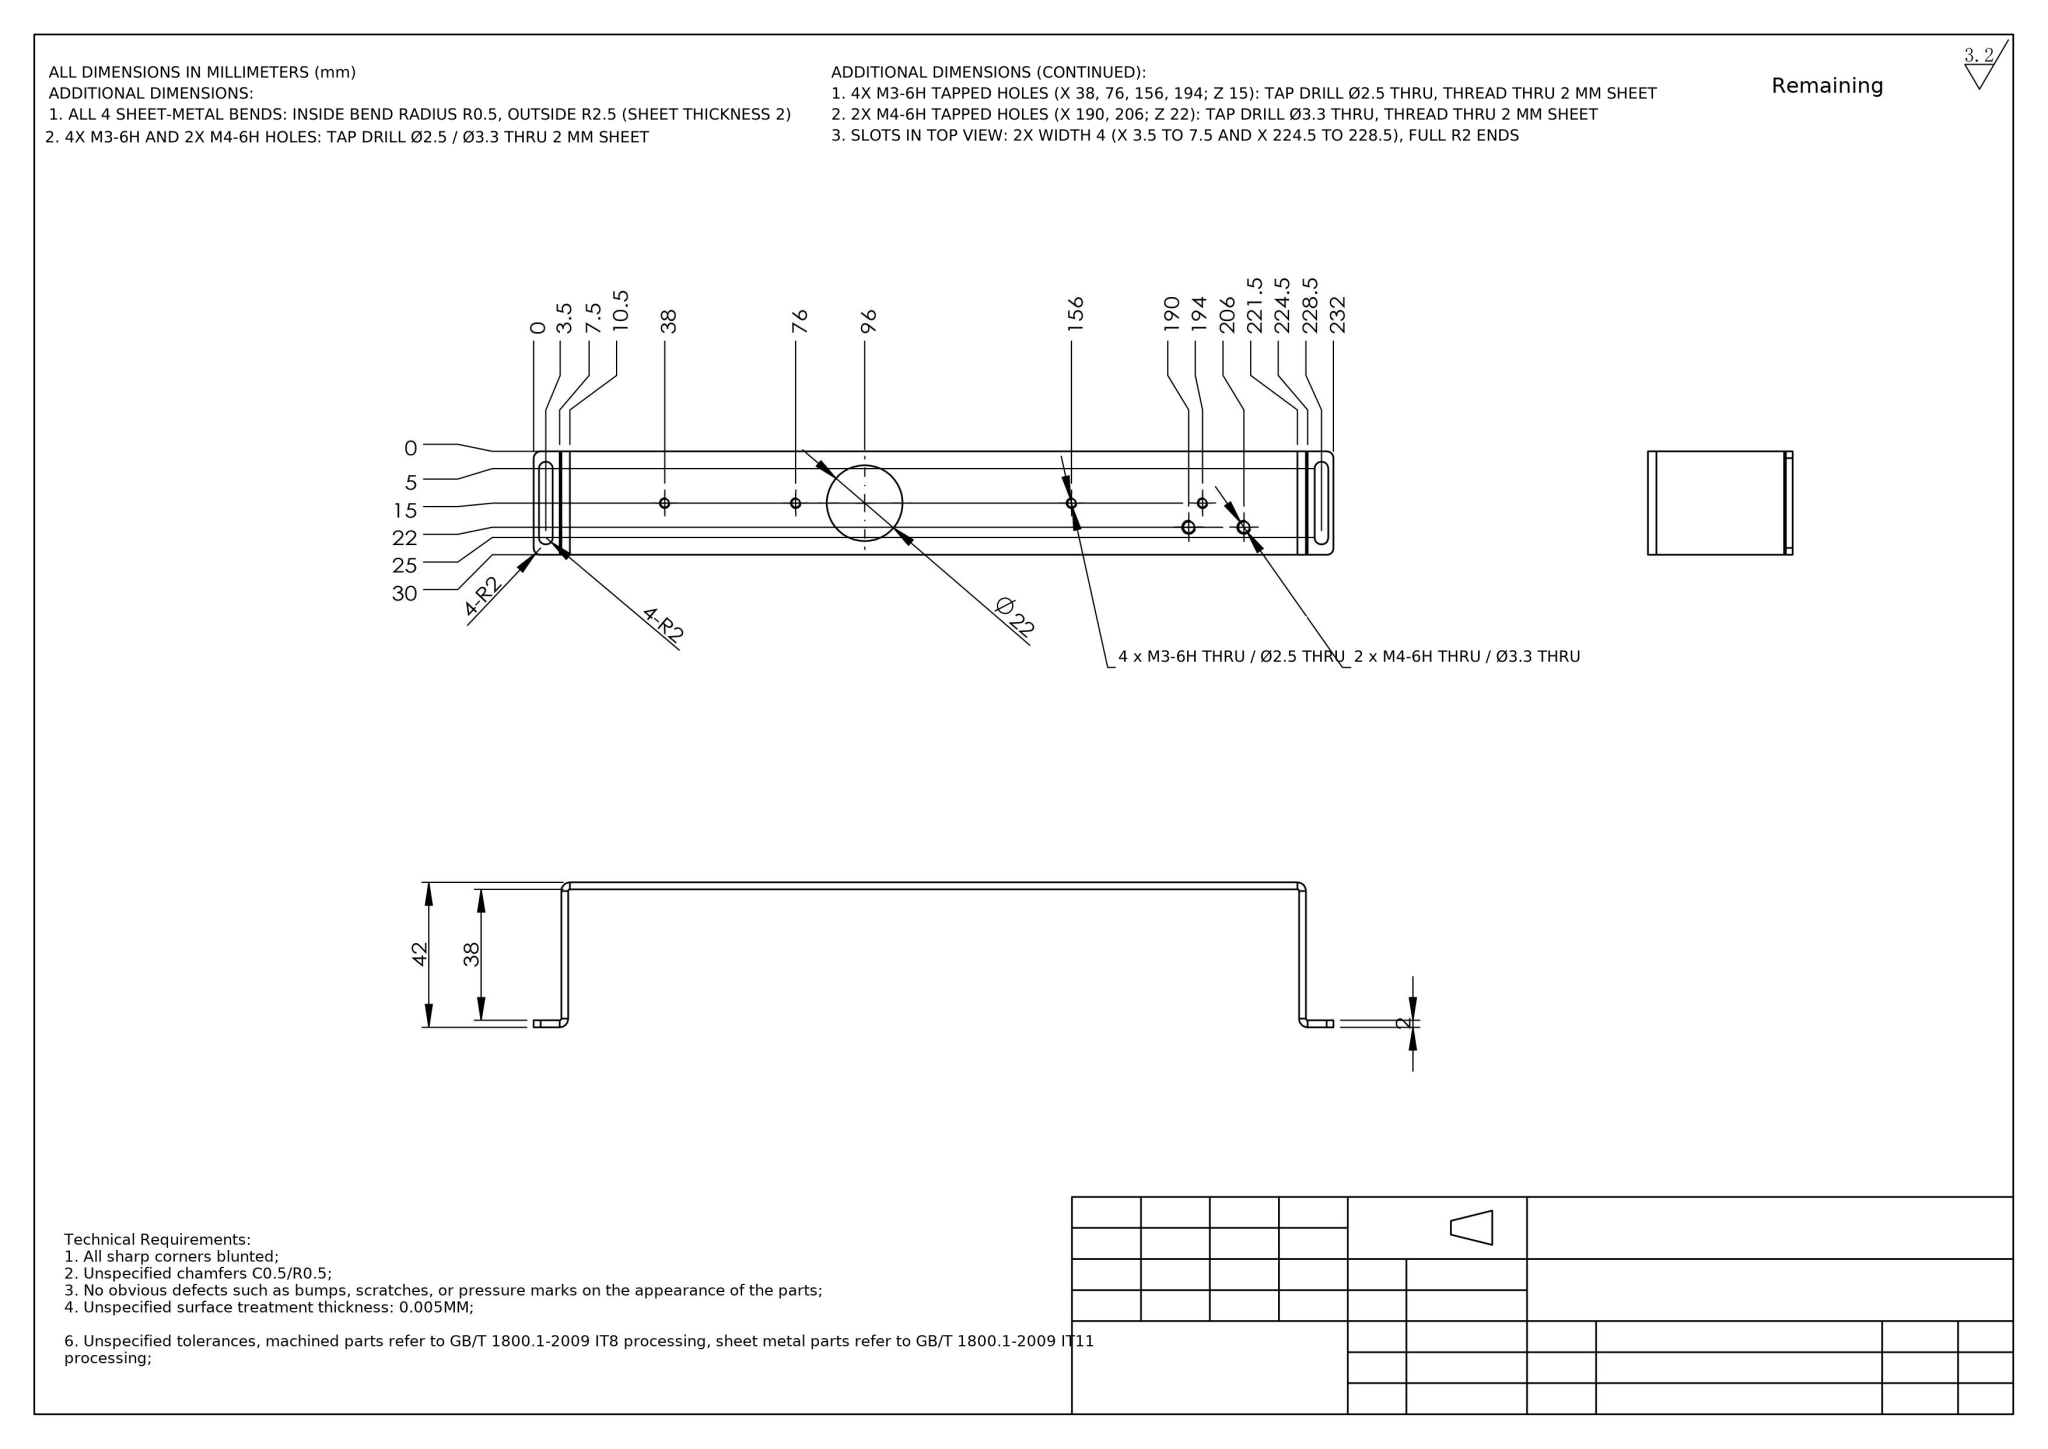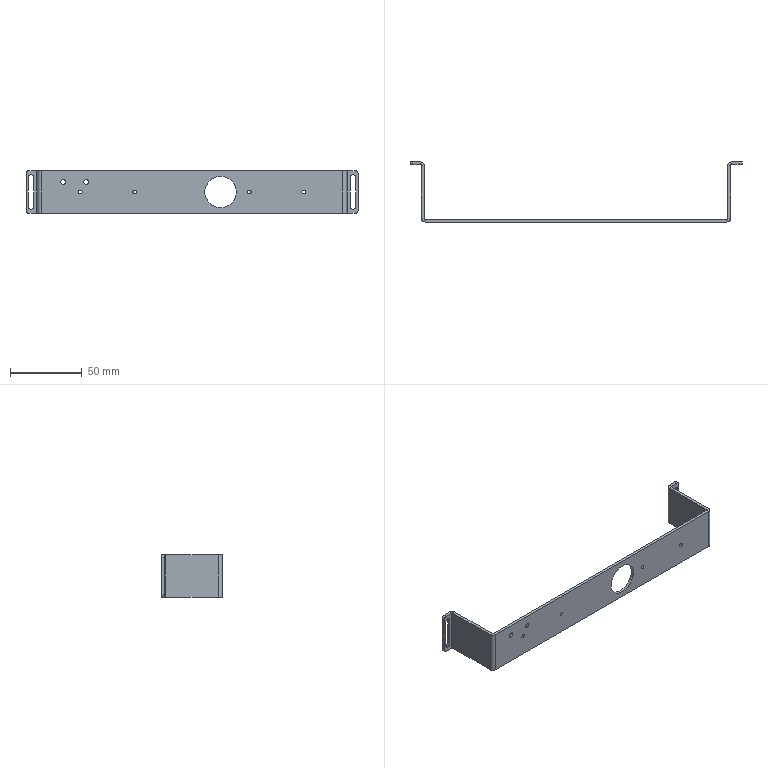Part | NX | mm | 1 solid | 66 faces | box 232 x 42 x 30 mm | volume 17355 mm3 | plane 34 | cylinder 32 | commonest cylinder face diameters 4 x10 2.5 x8 3.3 x4 5 x4 1 x4 22 x2